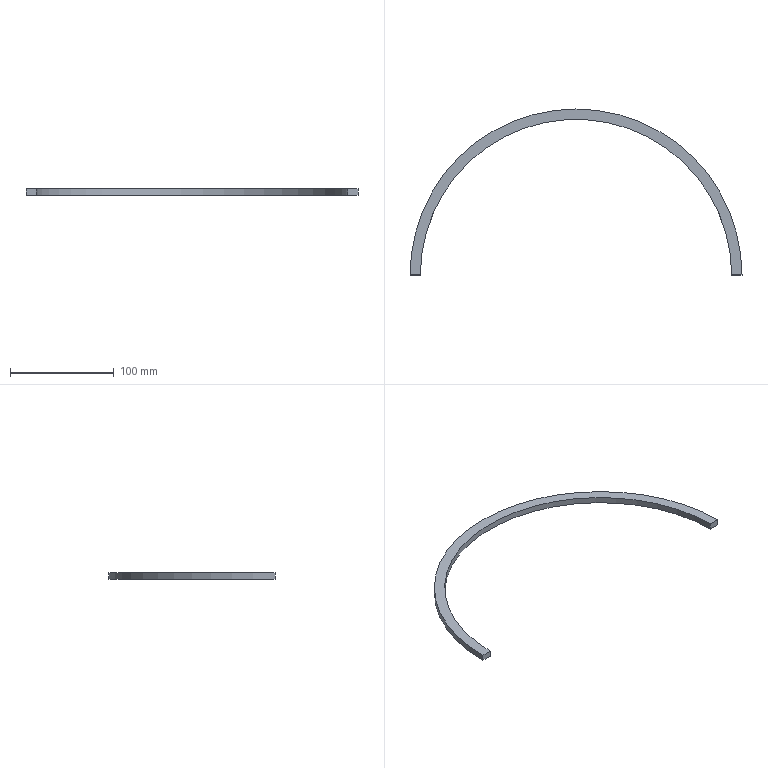Component | SolidWorks | JF21-80.1-1-3(_)-1-SOLID29-1 | 1 solid | 6 faces | box 320 x 160 x 6 mm | volume 29217 mm3 | plane 4 | cylinder 2 | commonest cylinder face diameters 320 x1 300 x1
STEP:
#1=COLOUR_RGB('',0.7922,0.8196,0.9333);
#2=FILL_AREA_STYLE_COLOUR('',#1);
#3=FILL_AREA_STYLE('',(#2));
#4=SURFACE_STYLE_FILL_AREA(#3);
#5=SURFACE_SIDE_STYLE('',(#4));
#6=SURFACE_STYLE_USAGE(.BOTH.,#5);
#7=PRESENTATION_STYLE_ASSIGNMENT((#6));
#8=CARTESIAN_POINT('',(6.299,-0.,12.559));
#9=VERTEX_POINT('',#8);
#10=CARTESIAN_POINT('',(-6.299,-0.,12.559));
#11=VERTEX_POINT('',#10);
#12=CARTESIAN_POINT('',(0.,0.,12.559));
#13=DIRECTION('',(0.,0.,1.));
#14=DIRECTION('',(1.,0.,0.));
#15=AXIS2_PLACEMENT_3D('',#12,#13,#14);
#16=CIRCLE('',#15,6.299);
#17=EDGE_CURVE('',#9,#11,#16,.T.);
#18=ORIENTED_EDGE('',*,*,#17,.T.);
#19=CARTESIAN_POINT('',(-6.299,-0.,12.795));
#20=VERTEX_POINT('',#19);
#21=CARTESIAN_POINT('',(-6.299,-0.,12.795));
#22=DIRECTION('',(0.,0.,1.));
#23=VECTOR('',#22,39.37);
#24=LINE('',#21,#23);
#25=EDGE_CURVE('',#11,#20,#24,.T.);
#26=ORIENTED_EDGE('',*,*,#25,.T.);
#27=CARTESIAN_POINT('',(6.299,-0.,12.795));
#28=VERTEX_POINT('',#27);
#29=CARTESIAN_POINT('',(0.,0.,12.795));
#30=DIRECTION('',(0.,0.,1.));
#31=DIRECTION('',(1.,0.,0.));
#32=AXIS2_PLACEMENT_3D('',#29,#30,#31);
#33=CIRCLE('',#32,6.299);
#34=EDGE_CURVE('',#28,#20,#33,.T.);
#35=ORIENTED_EDGE('',*,*,#34,.F.);
#36=CARTESIAN_POINT('',(6.299,-0.,12.795));
#37=DIRECTION('',(0.,0.,1.));
#38=VECTOR('',#37,39.37);
#39=LINE('',#36,#38);
#40=EDGE_CURVE('',#9,#28,#39,.T.);
#41=ORIENTED_EDGE('',*,*,#40,.F.);
#42=EDGE_LOOP('',(#18,#26,#35,#41));
#43=FACE_OUTER_BOUND('',#42,.T.);
#44=CARTESIAN_POINT('',(0.,0.,17.45));
#45=DIRECTION('',(0.,0.,1.));
#46=DIRECTION('',(-1.,0.,0.));
#47=AXIS2_PLACEMENT_3D('',#44,#45,#46);
#48=CYLINDRICAL_SURFACE('',#47,6.299);
#49=ADVANCED_FACE('',(#43),#48,.T.);
#50=CARTESIAN_POINT('',(5.906,-0.,12.559));
#51=VERTEX_POINT('',#50);
#52=CARTESIAN_POINT('',(-5.906,-0.,12.559));
#53=VERTEX_POINT('',#52);
#54=CARTESIAN_POINT('',(0.,0.,12.559));
#55=DIRECTION('',(0.,0.,1.));
#56=DIRECTION('',(1.,0.,0.));
#57=AXIS2_PLACEMENT_3D('',#54,#55,#56);
#58=CIRCLE('',#57,5.906);
#59=EDGE_CURVE('',#51,#53,#58,.T.);
#60=ORIENTED_EDGE('',*,*,#59,.T.);
#61=CARTESIAN_POINT('',(-6.299,-0.,12.559));
#62=DIRECTION('',(-1.,-0.,0.));
#63=VECTOR('',#62,39.37);
#64=LINE('',#61,#63);
#65=EDGE_CURVE('',#53,#11,#64,.T.);
#66=ORIENTED_EDGE('',*,*,#65,.T.);
#67=ORIENTED_EDGE('',*,*,#17,.F.);
#68=CARTESIAN_POINT('',(6.299,-0.,12.559));
#69=DIRECTION('',(1.,-0.,0.));
#70=VECTOR('',#69,39.37);
#71=LINE('',#68,#70);
#72=EDGE_CURVE('',#51,#9,#71,.T.);
#73=ORIENTED_EDGE('',*,*,#72,.F.);
#74=EDGE_LOOP('',(#60,#66,#67,#73));
#75=FACE_OUTER_BOUND('',#74,.T.);
#76=CARTESIAN_POINT('',(6.299,-0.,12.559));
#77=DIRECTION('',(0.,0.,1.));
#78=DIRECTION('',(-1.,0.,0.));
#79=AXIS2_PLACEMENT_3D('',#76,#77,#78);
#80=PLANE('',#79);
#81=ADVANCED_FACE('',(#75),#80,.F.);
#82=CARTESIAN_POINT('',(5.906,-0.,12.795));
#83=VERTEX_POINT('',#82);
#84=CARTESIAN_POINT('',(-5.906,-0.,12.795));
#85=VERTEX_POINT('',#84);
#86=CARTESIAN_POINT('',(0.,0.,12.795));
#87=DIRECTION('',(0.,0.,1.));
#88=DIRECTION('',(1.,0.,0.));
#89=AXIS2_PLACEMENT_3D('',#86,#87,#88);
#90=CIRCLE('',#89,5.906);
#91=EDGE_CURVE('',#83,#85,#90,.T.);
#92=ORIENTED_EDGE('',*,*,#91,.T.);
#93=CARTESIAN_POINT('',(-5.906,-0.,12.559));
#94=DIRECTION('',(0.,0.,-1.));
#95=VECTOR('',#94,39.37);
#96=LINE('',#93,#95);
#97=EDGE_CURVE('',#85,#53,#96,.T.);
#98=ORIENTED_EDGE('',*,*,#97,.T.);
#99=ORIENTED_EDGE('',*,*,#59,.F.);
#100=CARTESIAN_POINT('',(5.906,-0.,12.559));
#101=DIRECTION('',(0.,0.,-1.));
#102=VECTOR('',#101,39.37);
#103=LINE('',#100,#102);
#104=EDGE_CURVE('',#83,#51,#103,.T.);
#105=ORIENTED_EDGE('',*,*,#104,.F.);
#106=EDGE_LOOP('',(#92,#98,#99,#105));
#107=FACE_OUTER_BOUND('',#106,.T.);
#108=CARTESIAN_POINT('',(0.,0.,17.45));
#109=DIRECTION('',(0.,0.,1.));
#110=DIRECTION('',(-1.,0.,0.));
#111=AXIS2_PLACEMENT_3D('',#108,#109,#110);
#112=CYLINDRICAL_SURFACE('',#111,5.906);
#113=ADVANCED_FACE('',(#107),#112,.F.);
#114=ORIENTED_EDGE('',*,*,#40,.T.);
#115=CARTESIAN_POINT('',(5.906,-0.,12.795));
#116=DIRECTION('',(-1.,0.,-0.));
#117=VECTOR('',#116,39.37);
#118=LINE('',#115,#117);
#119=EDGE_CURVE('',#28,#83,#118,.T.);
#120=ORIENTED_EDGE('',*,*,#119,.T.);
#121=ORIENTED_EDGE('',*,*,#104,.T.);
#122=ORIENTED_EDGE('',*,*,#72,.T.);
#123=EDGE_LOOP('',(#114,#120,#121,#122));
#124=FACE_OUTER_BOUND('',#123,.T.);
#125=CARTESIAN_POINT('',(6.299,-0.,12.559));
#126=DIRECTION('',(0.,1.,0.));
#127=DIRECTION('',(0.,0.,-1.));
#128=AXIS2_PLACEMENT_3D('',#125,#126,#127);
#129=PLANE('',#128);
#130=ADVANCED_FACE('',(#124),#129,.F.);
#131=ORIENTED_EDGE('',*,*,#119,.F.);
#132=ORIENTED_EDGE('',*,*,#34,.T.);
#133=CARTESIAN_POINT('',(-5.906,-0.,12.795));
#134=DIRECTION('',(1.,0.,-0.));
#135=VECTOR('',#134,39.37);
#136=LINE('',#133,#135);
#137=EDGE_CURVE('',#20,#85,#136,.T.);
#138=ORIENTED_EDGE('',*,*,#137,.T.);
#139=ORIENTED_EDGE('',*,*,#91,.F.);
#140=EDGE_LOOP('',(#131,#132,#138,#139));
#141=FACE_OUTER_BOUND('',#140,.T.);
#142=CARTESIAN_POINT('',(5.906,-0.,12.795));
#143=DIRECTION('',(0.,0.,-1.));
#144=DIRECTION('',(1.,0.,0.));
#145=AXIS2_PLACEMENT_3D('',#142,#143,#144);
#146=PLANE('',#145);
#147=ADVANCED_FACE('',(#141),#146,.F.);
#148=ORIENTED_EDGE('',*,*,#25,.F.);
#149=ORIENTED_EDGE('',*,*,#65,.F.);
#150=ORIENTED_EDGE('',*,*,#97,.F.);
#151=ORIENTED_EDGE('',*,*,#137,.F.);
#152=EDGE_LOOP('',(#148,#149,#150,#151));
#153=FACE_OUTER_BOUND('',#152,.T.);
#154=CARTESIAN_POINT('',(-6.299,-0.,12.559));
#155=DIRECTION('',(0.,-1.,0.));
#156=DIRECTION('',(0.,0.,-1.));
#157=AXIS2_PLACEMENT_3D('',#154,#155,#156);
#158=PLANE('',#157);
#159=ADVANCED_FACE('',(#153),#158,.T.);
#160=CLOSED_SHELL('',(#49,#81,#113,#130,#147,#159));
#161=MANIFOLD_SOLID_BREP('',#160);
#162=STYLED_ITEM('',(#7),#161);
#163=(LENGTH_UNIT()NAMED_UNIT(*)SI_UNIT($,.METRE.));
#164=LENGTH_MEASURE_WITH_UNIT(LENGTH_MEASURE(0.0254),#163);
#165=DIMENSIONAL_EXPONENTS(1.,0.,0.,0.,0.,0.,0.);
#166=(CONVERSION_BASED_UNIT('',#164)LENGTH_UNIT()NAMED_UNIT(#165));
#167=UNCERTAINTY_MEASURE_WITH_UNIT(LENGTH_MEASURE(0.00001),#166,'','');
#168=(NAMED_UNIT(*)PLANE_ANGLE_UNIT()SI_UNIT($,.RADIAN.));
#169=(NAMED_UNIT(*)SI_UNIT($,.STERADIAN.)SOLID_ANGLE_UNIT());
#170=(GEOMETRIC_REPRESENTATION_CONTEXT(3)GLOBAL_UNCERTAINTY_ASSIGNED_CONTEXT((#167))GLOBAL_UNIT_ASSIGNED_CONTEXT((#166,#168,#169))REPRESENTATION_CONTEXT('',''));
#171=MECHANICAL_DESIGN_GEOMETRIC_PRESENTATION_REPRESENTATION('',(#162),#170);
#172=PRESENTATION_LAYER_ASSIGNMENT('','',(#162));
#173=CARTESIAN_POINT('',(0.,0.,0.));
#174=DIRECTION('',(0.,0.,1.));
#175=DIRECTION('',(1.,0.,0.));
#176=AXIS2_PLACEMENT_3D('',#173,#174,#175);
#177=(LENGTH_UNIT()NAMED_UNIT(*)SI_UNIT($,.METRE.));
#178=LENGTH_MEASURE_WITH_UNIT(LENGTH_MEASURE(0.0254),#177);
#179=DIMENSIONAL_EXPONENTS(1.,0.,0.,0.,0.,0.,0.);
#180=(CONVERSION_BASED_UNIT('',#178)LENGTH_UNIT()NAMED_UNIT(#179));
#181=UNCERTAINTY_MEASURE_WITH_UNIT(LENGTH_MEASURE(0.00001),#180,'','');
#182=(NAMED_UNIT(*)PLANE_ANGLE_UNIT()SI_UNIT($,.RADIAN.));
#183=(NAMED_UNIT(*)SI_UNIT($,.STERADIAN.)SOLID_ANGLE_UNIT());
#184=(GEOMETRIC_REPRESENTATION_CONTEXT(3)GLOBAL_UNCERTAINTY_ASSIGNED_CONTEXT((#181))GLOBAL_UNIT_ASSIGNED_CONTEXT((#180,#182,#183))REPRESENTATION_CONTEXT('',''));
#185=ADVANCED_BREP_SHAPE_REPRESENTATION('',(#161,#176),#184);